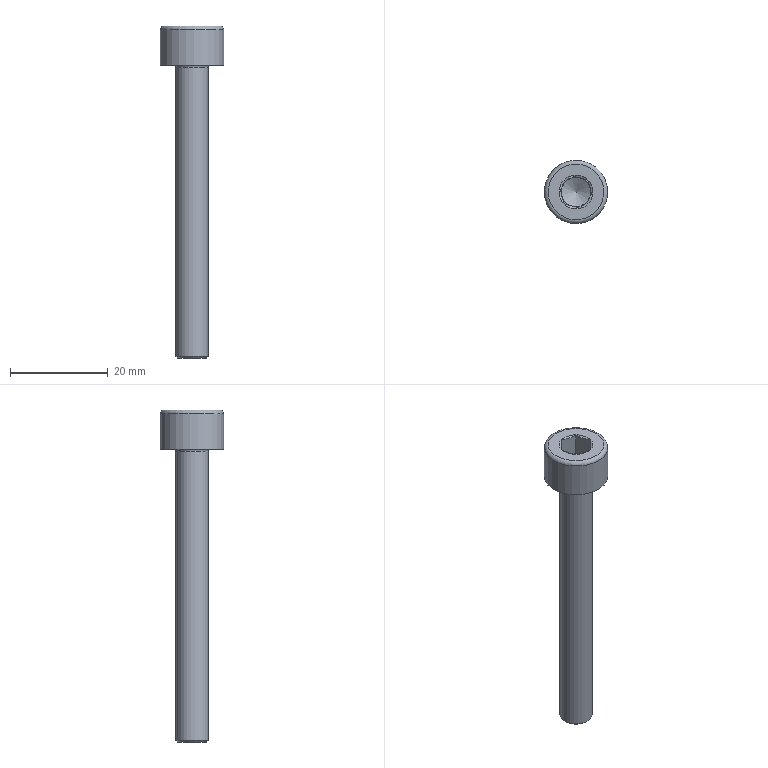Component | NX | SCREW_M8X60_5 | 1 solid | 27 faces | volume 2957 mm3 | plane 15 | cone 8 | cylinder 2 | torus 2 | commonest cylinder face diameters 6.619 x1 13 x1